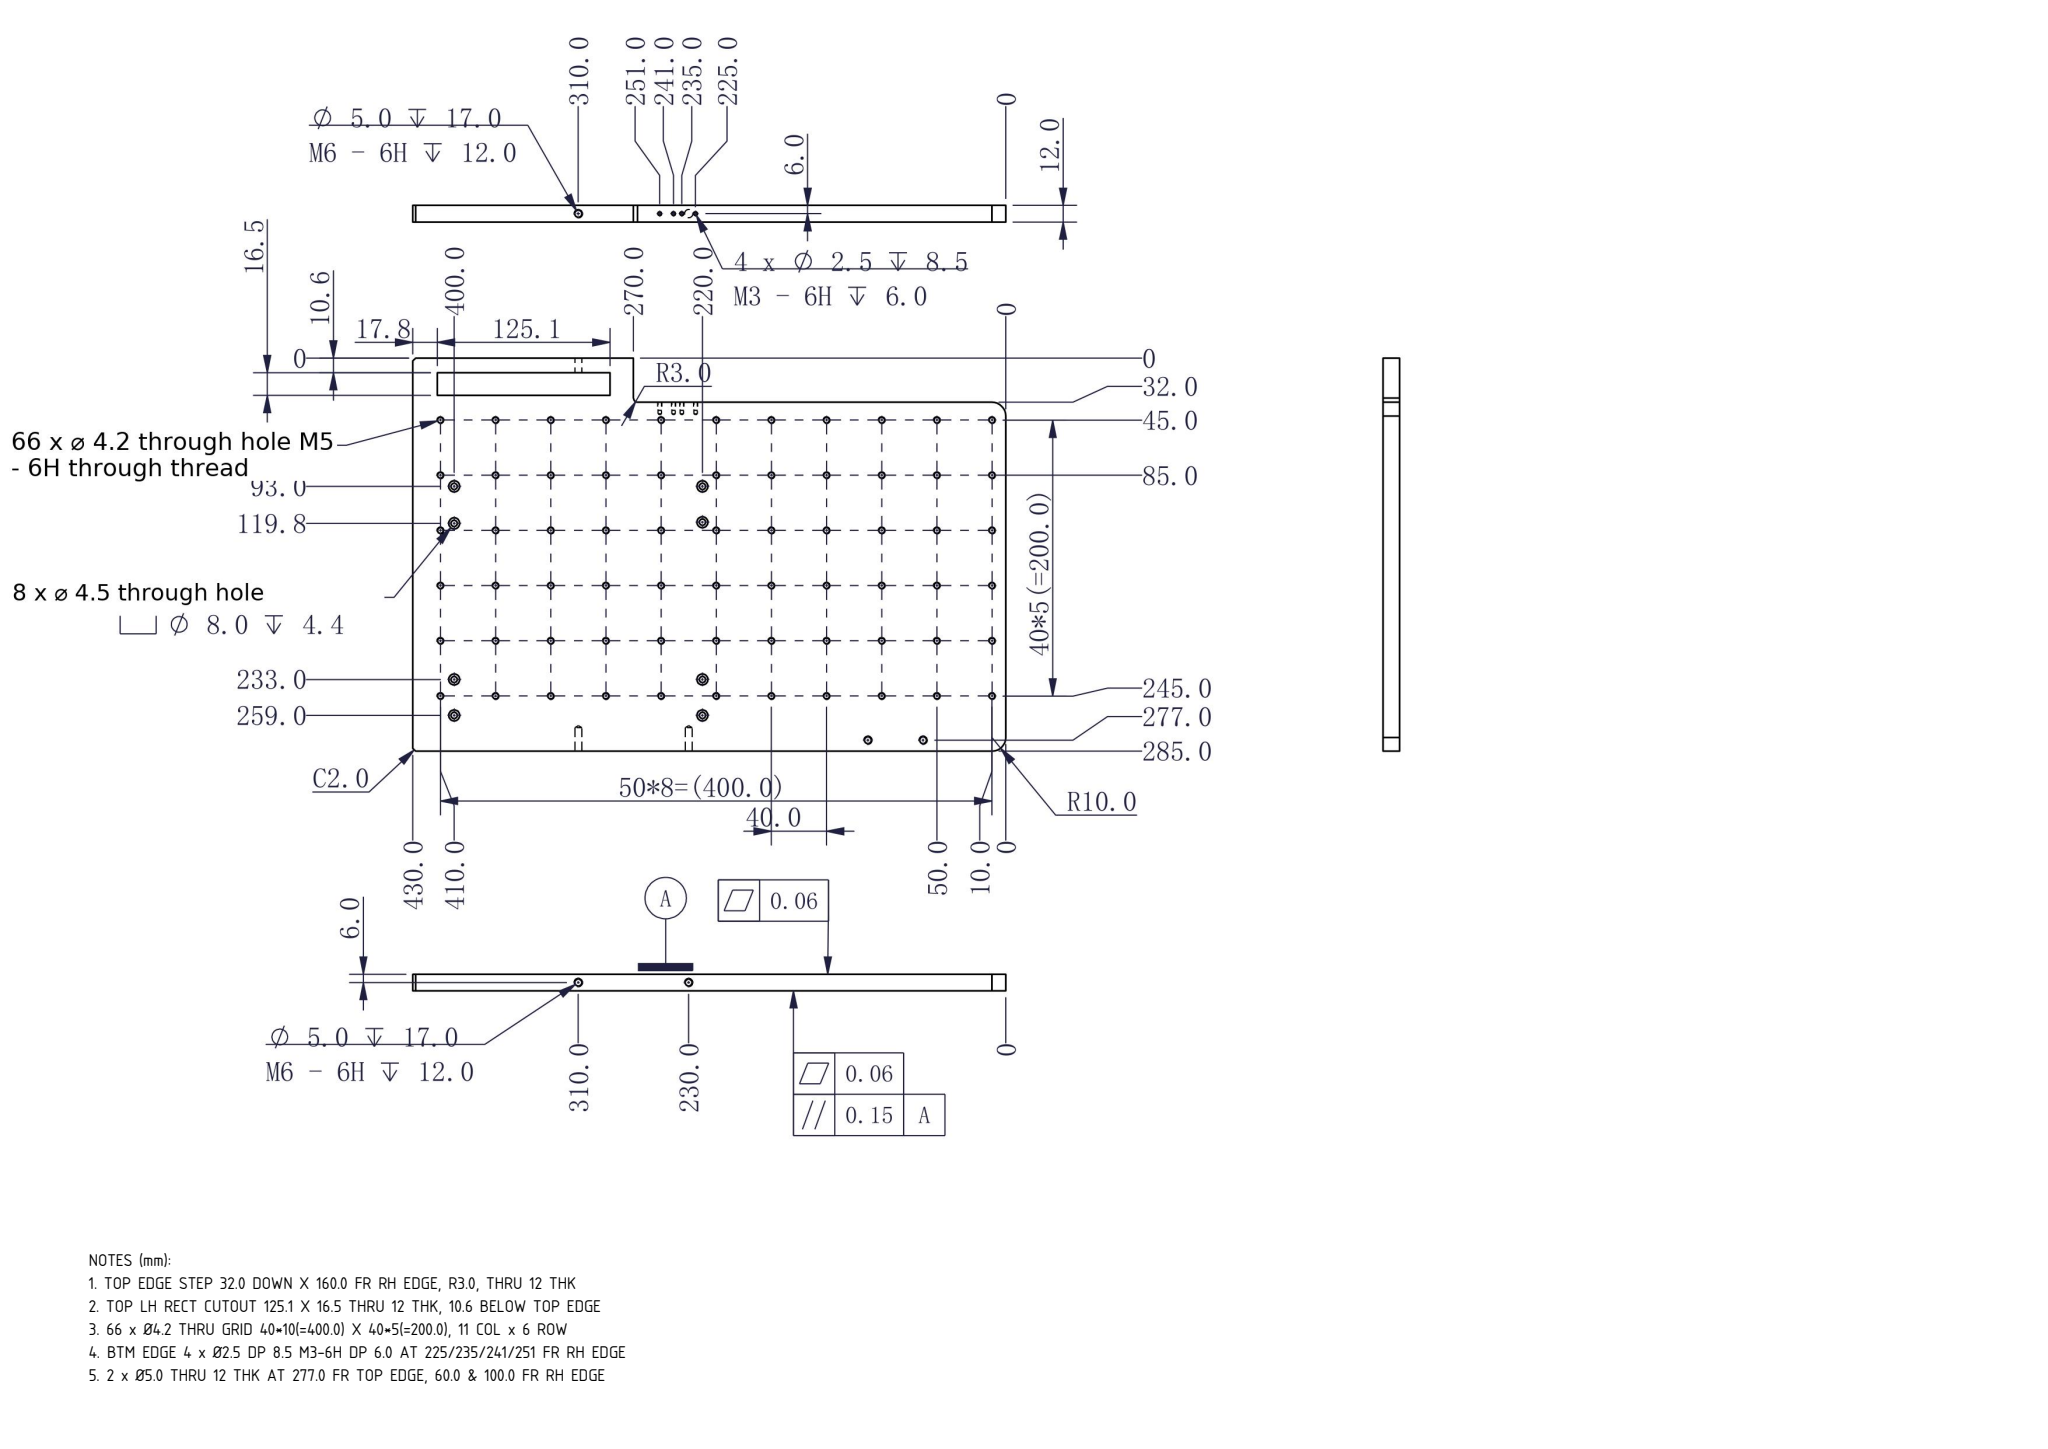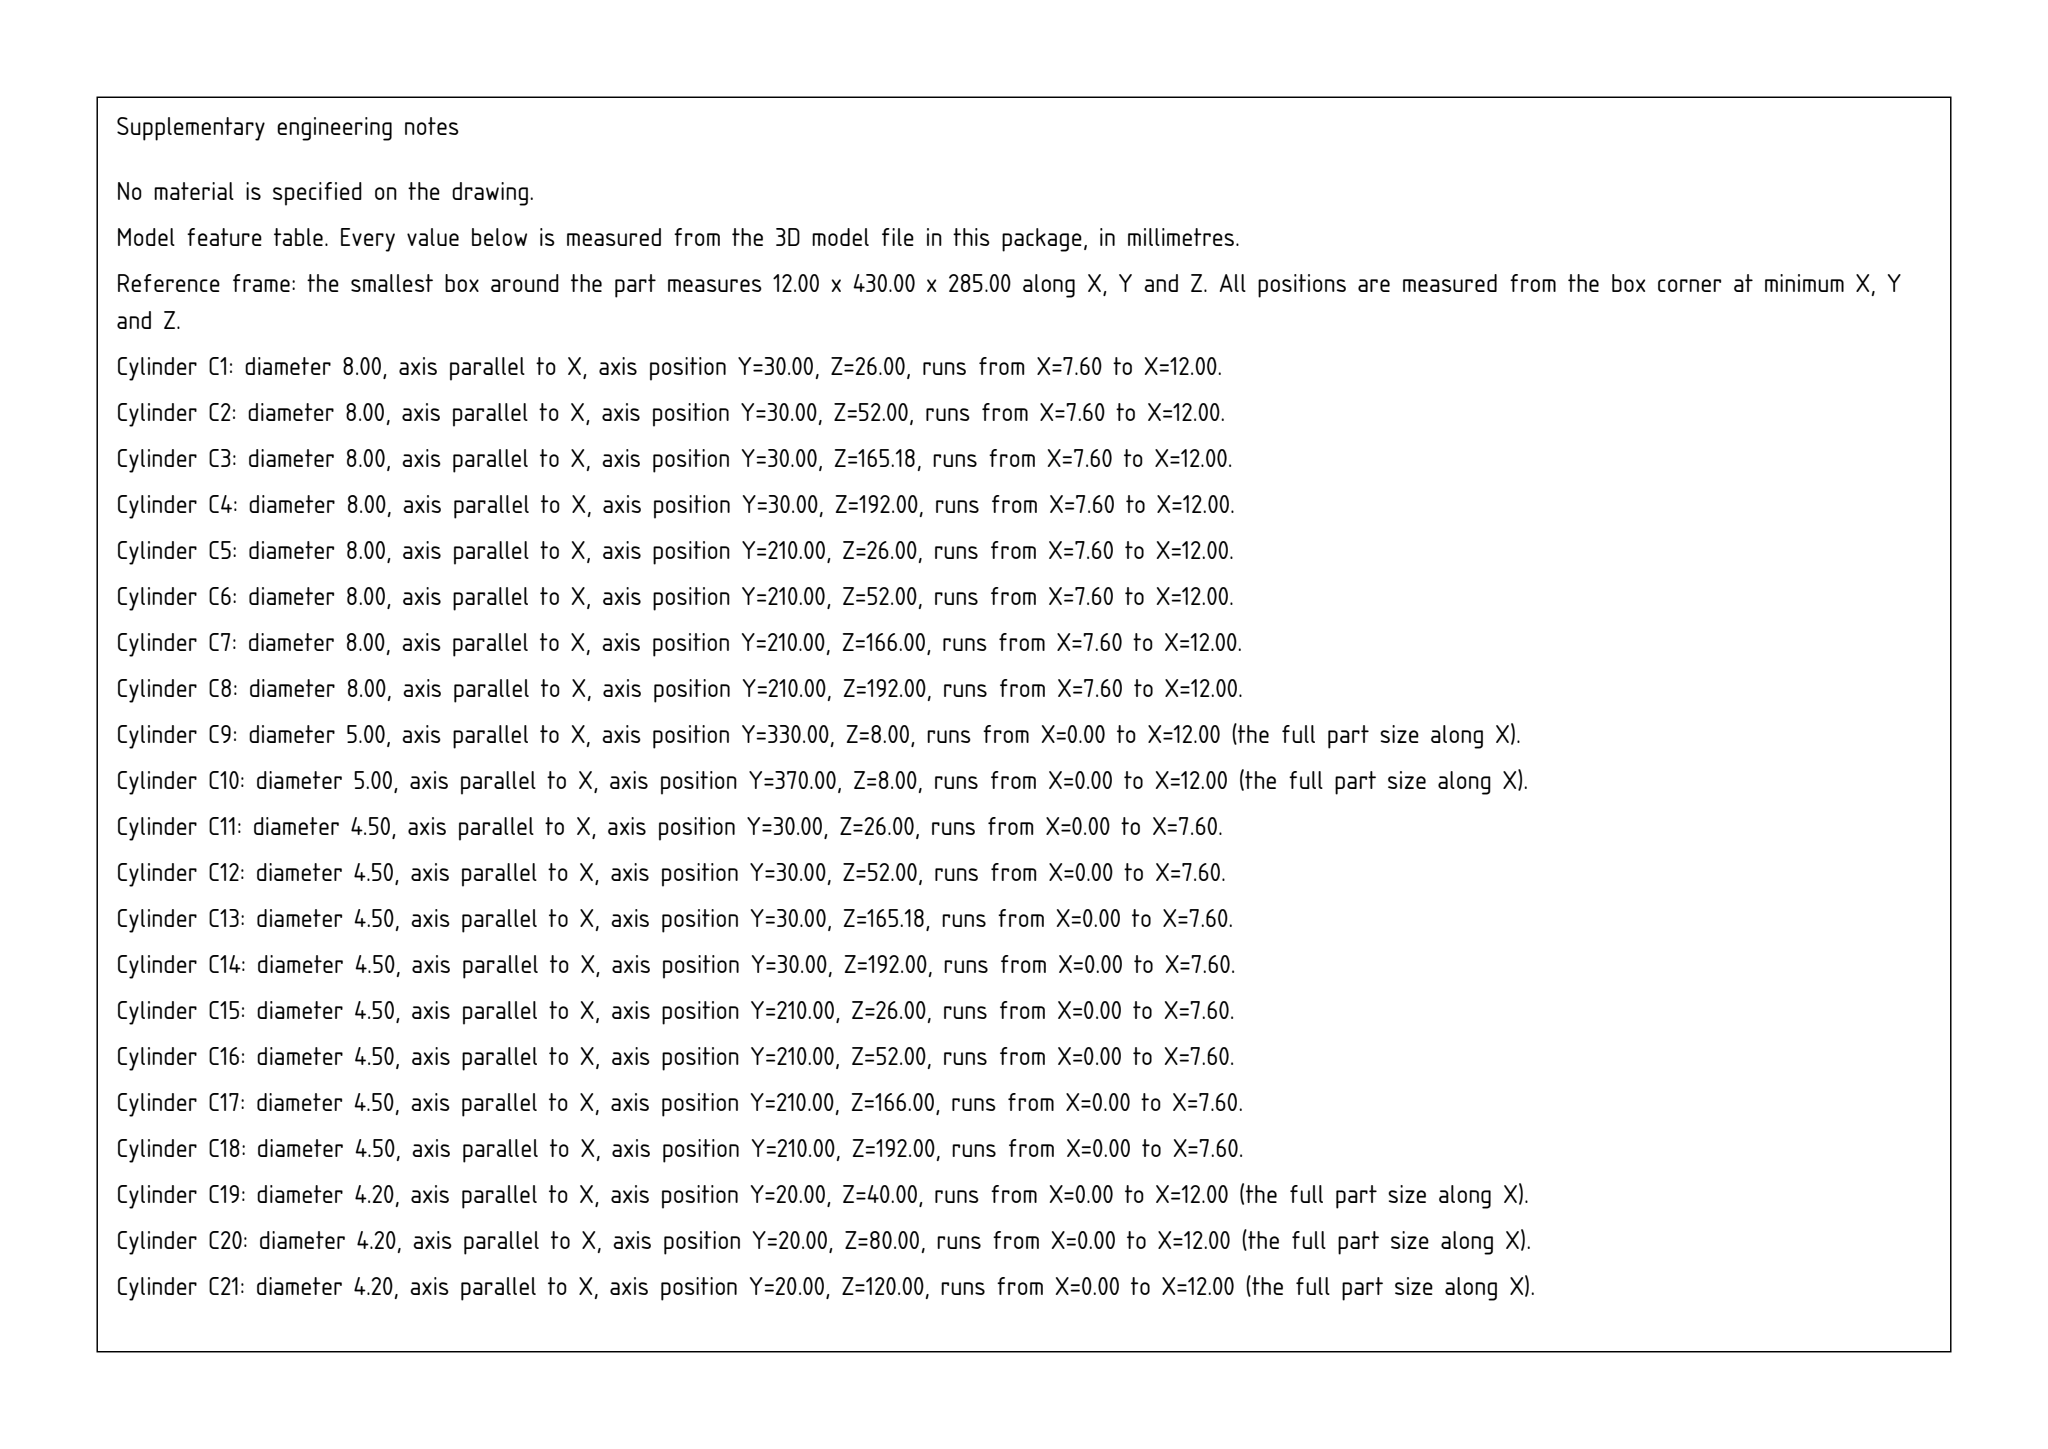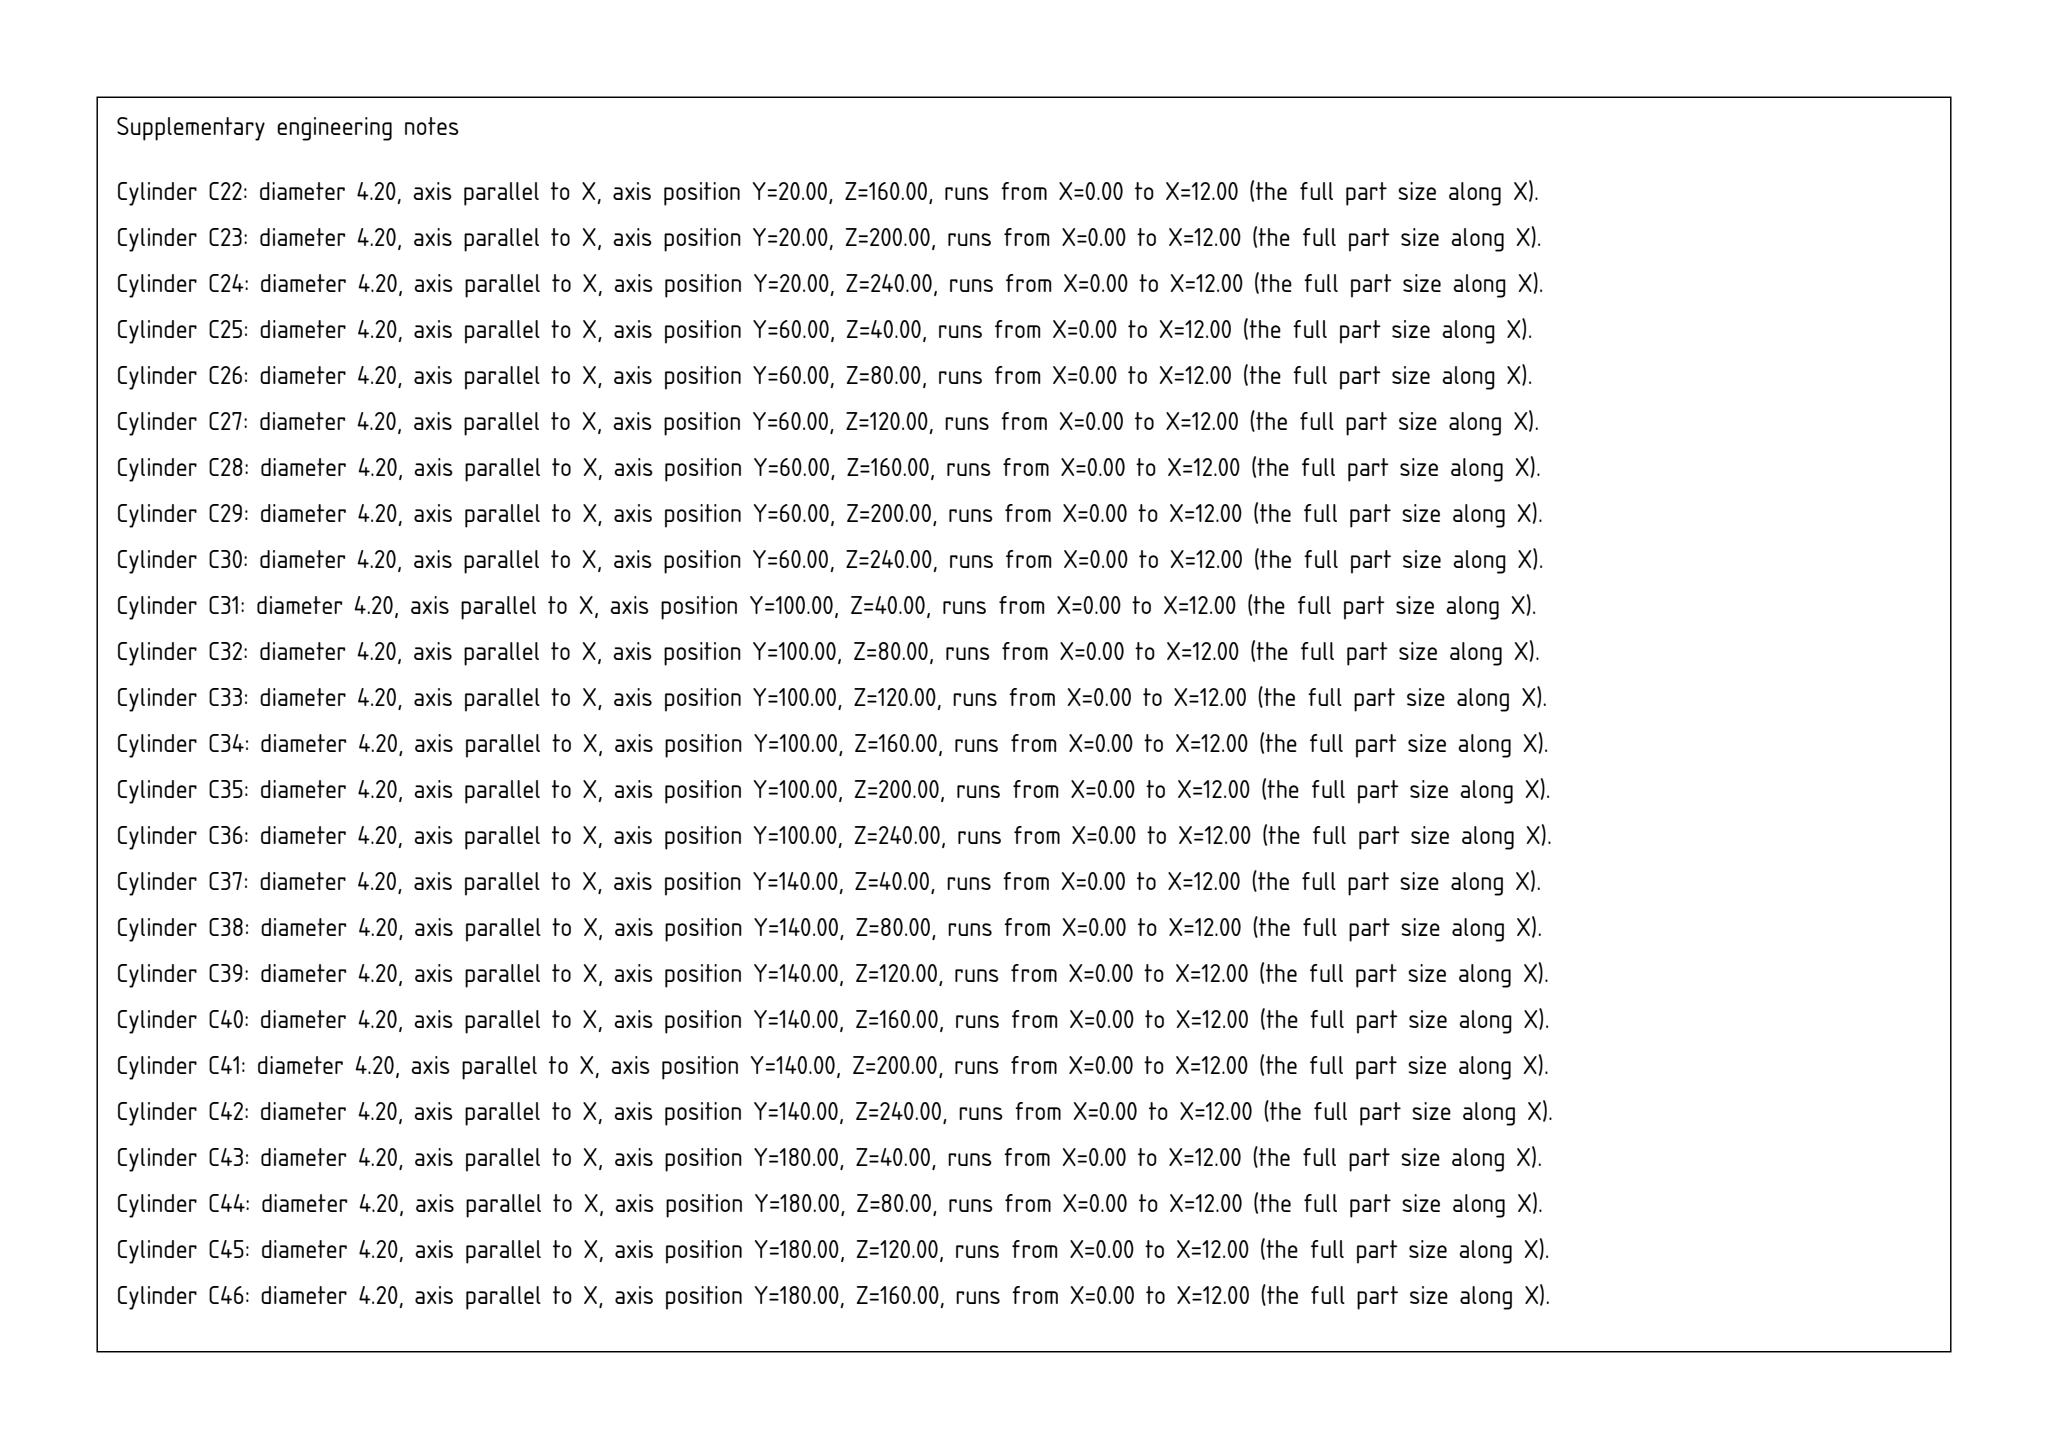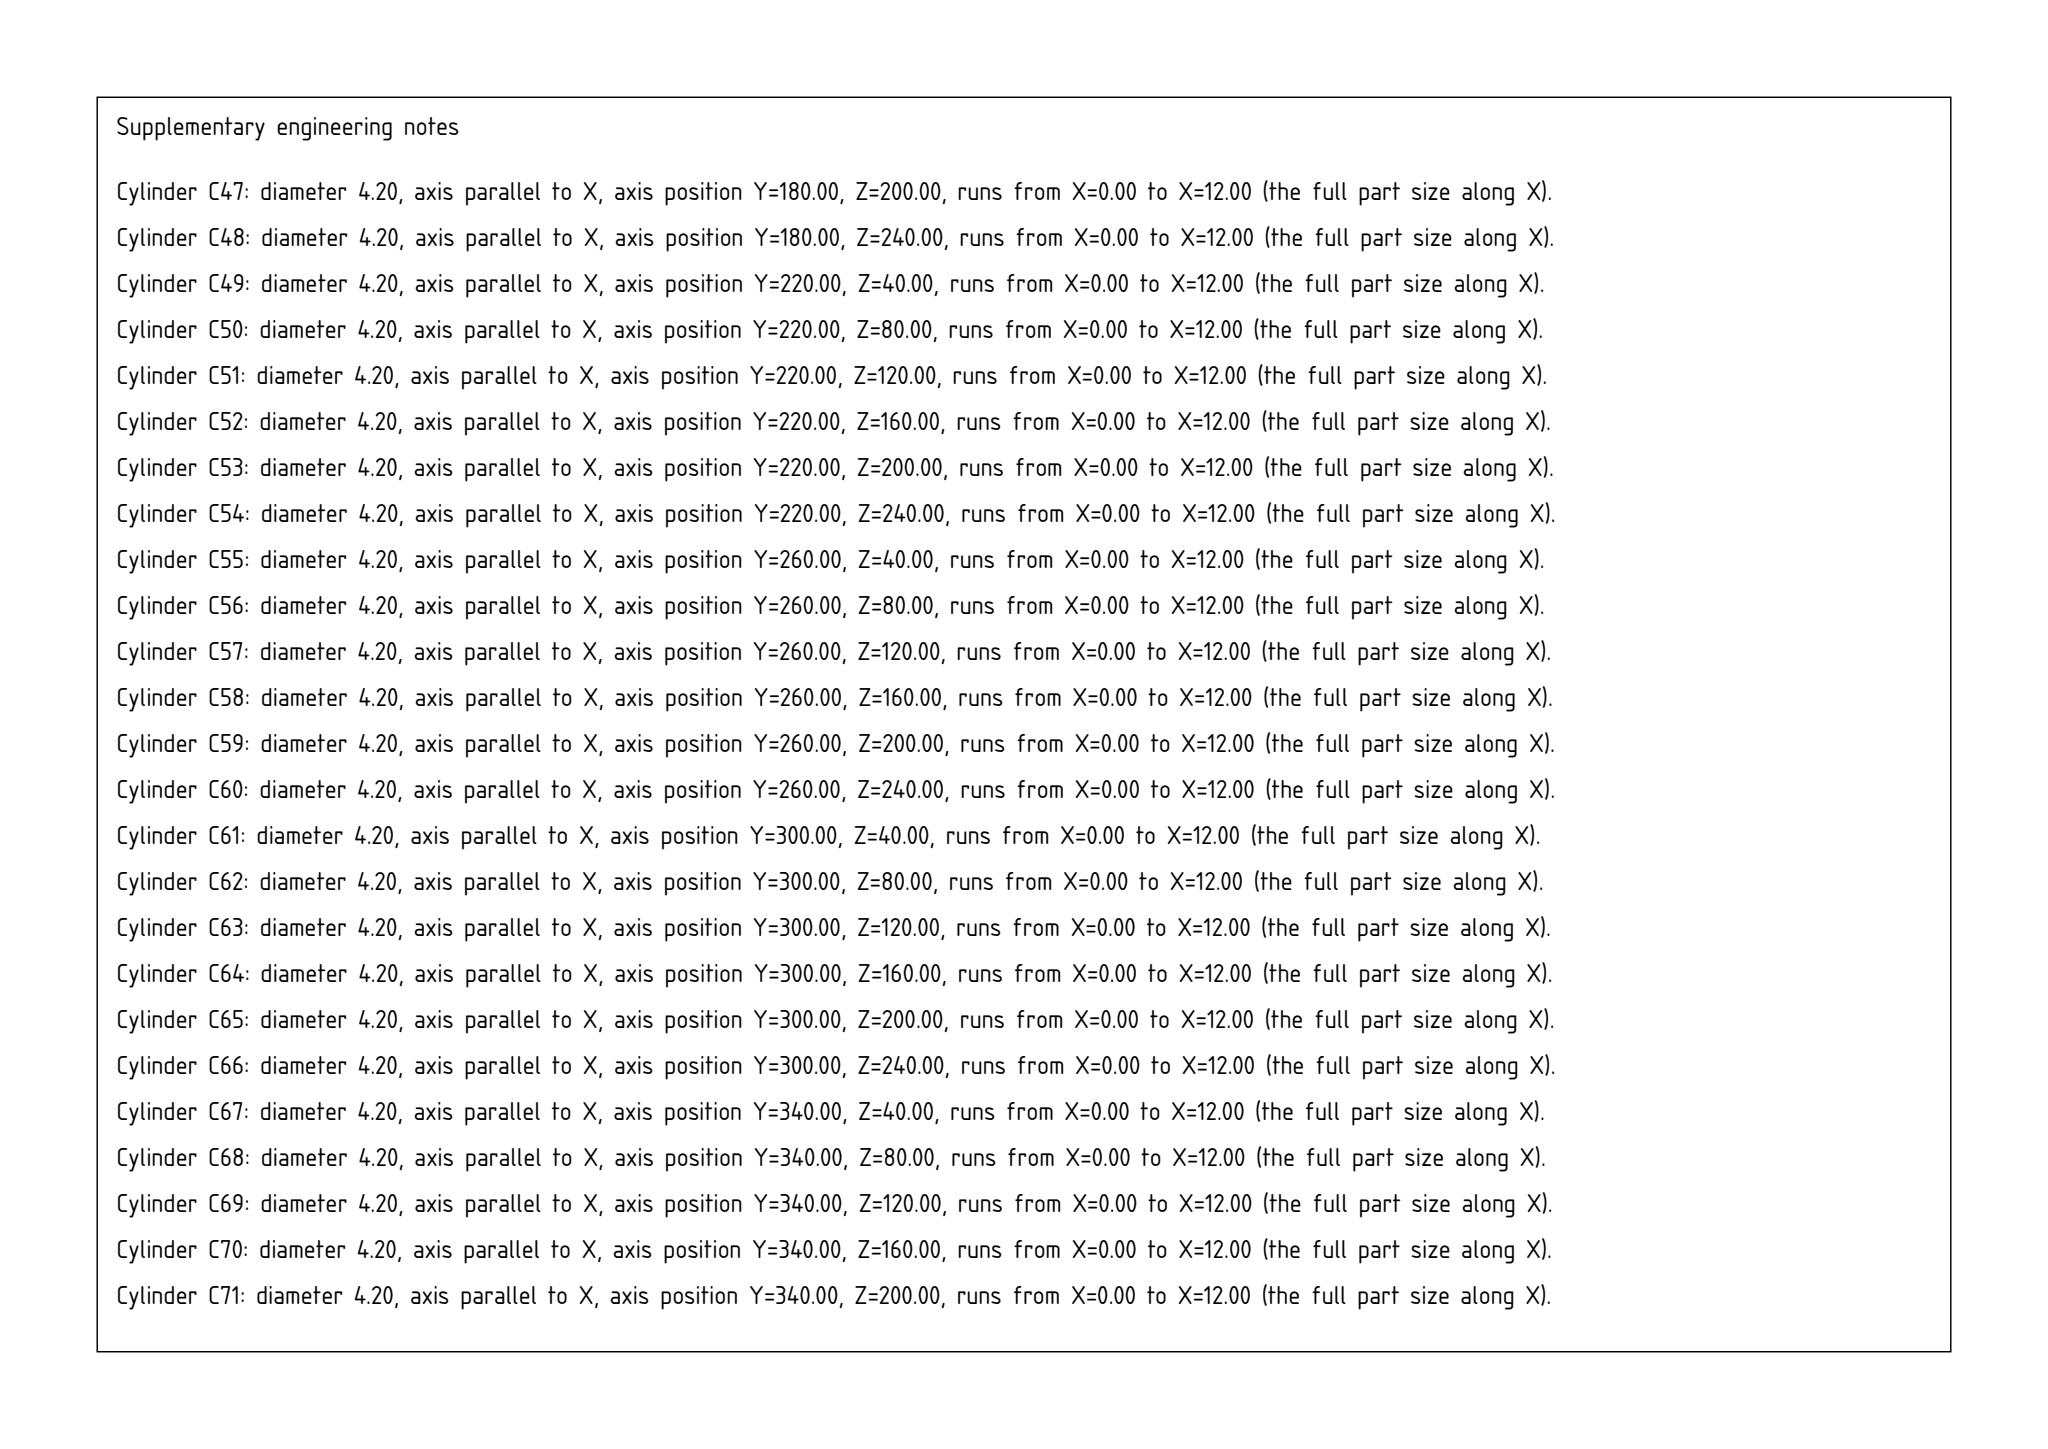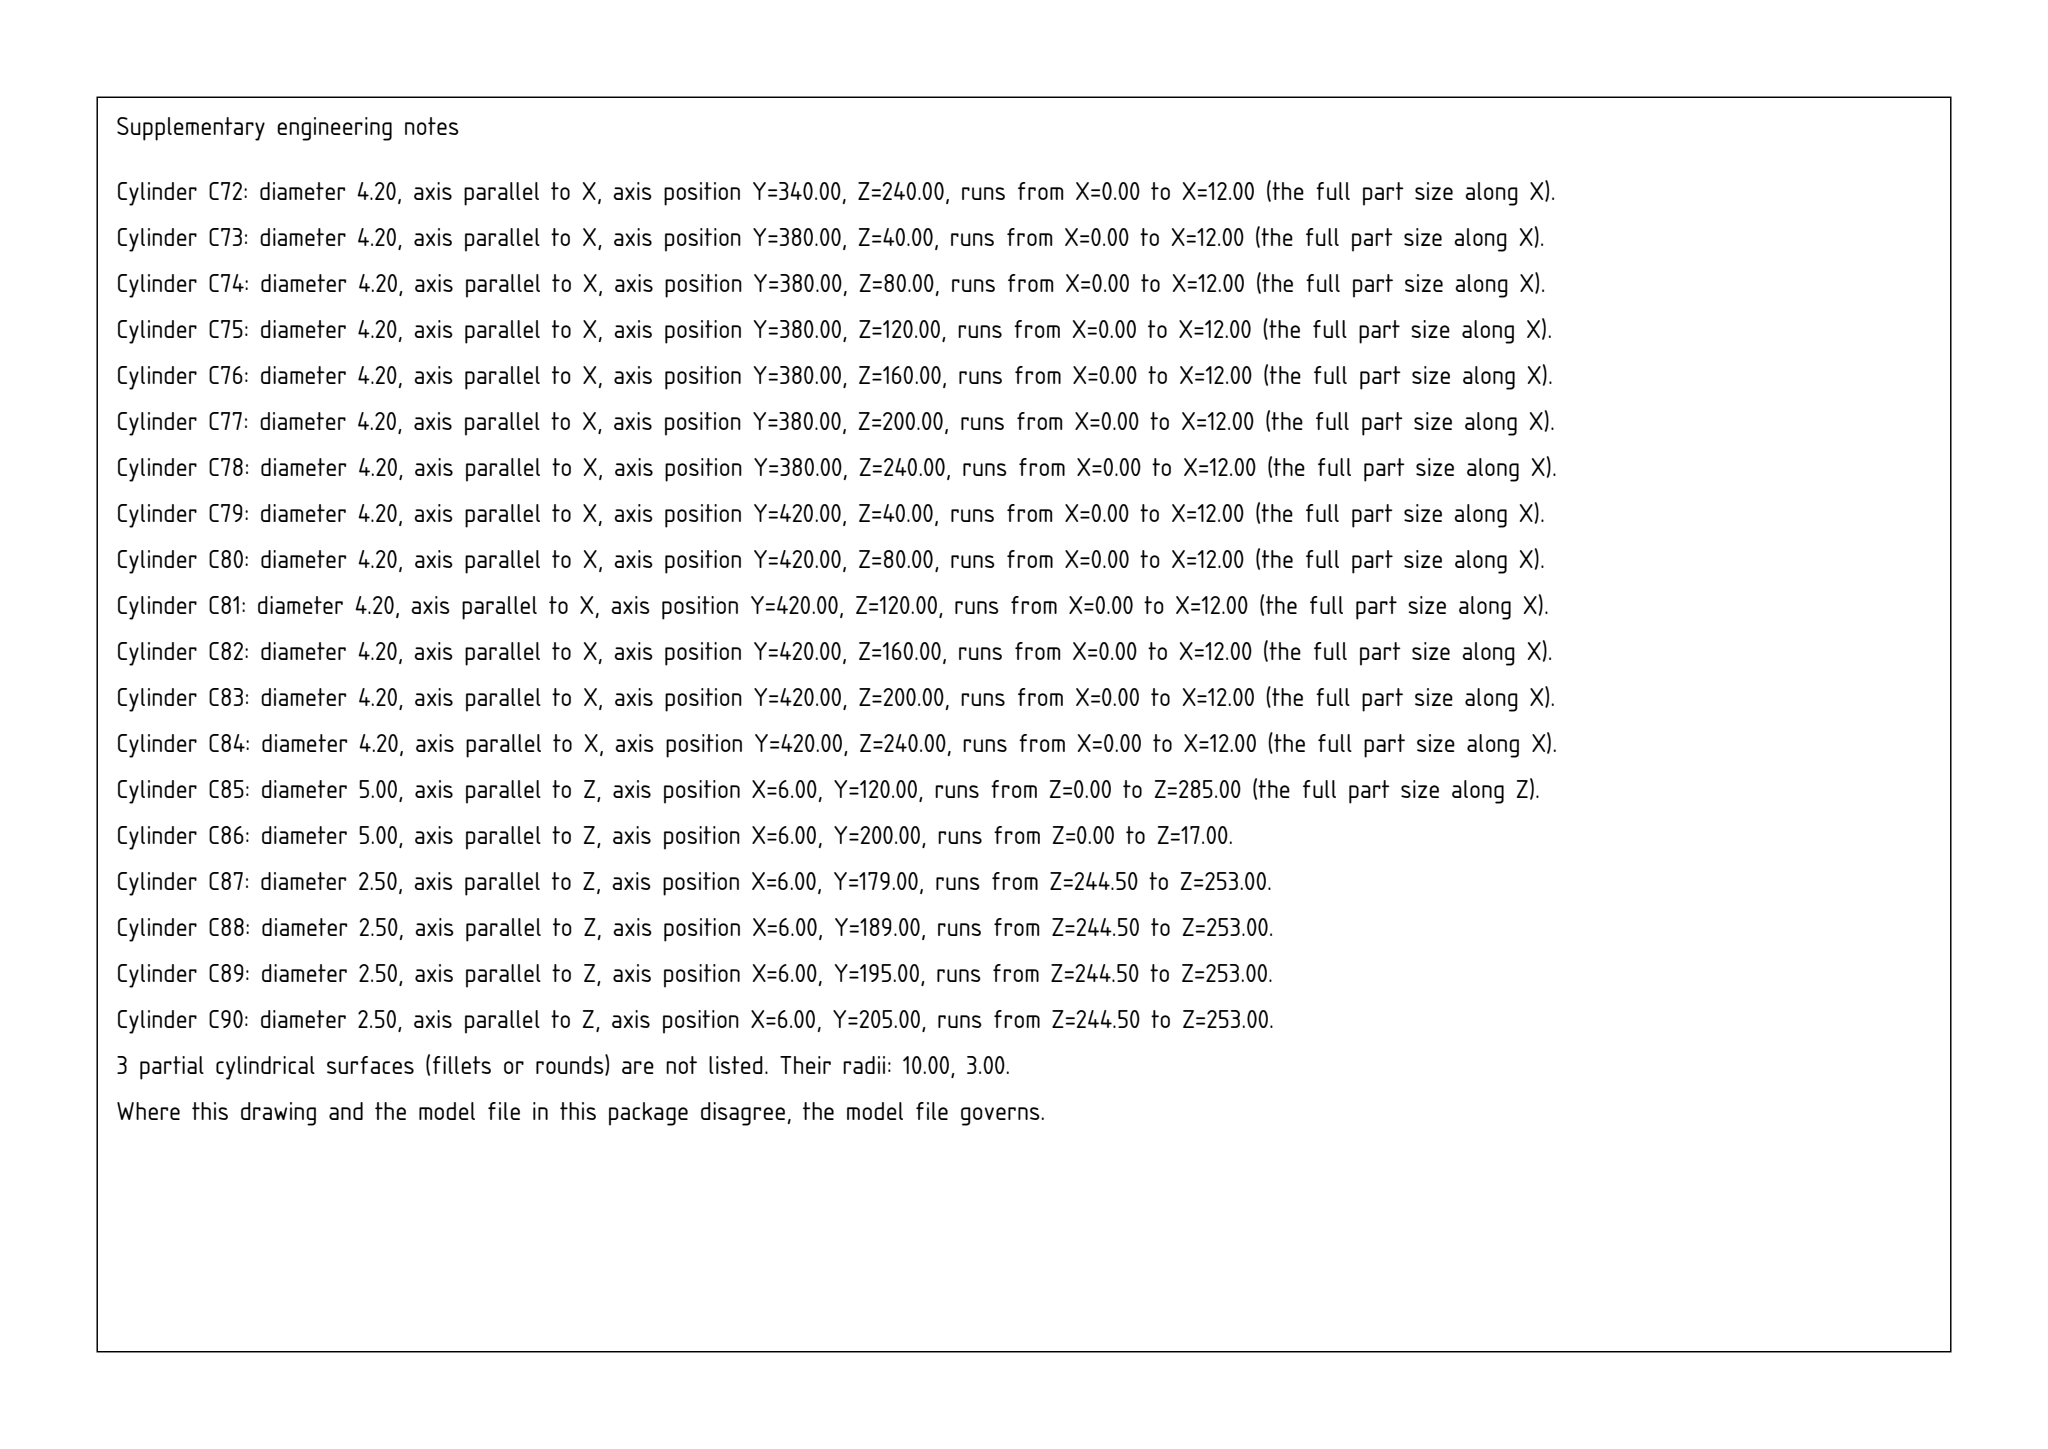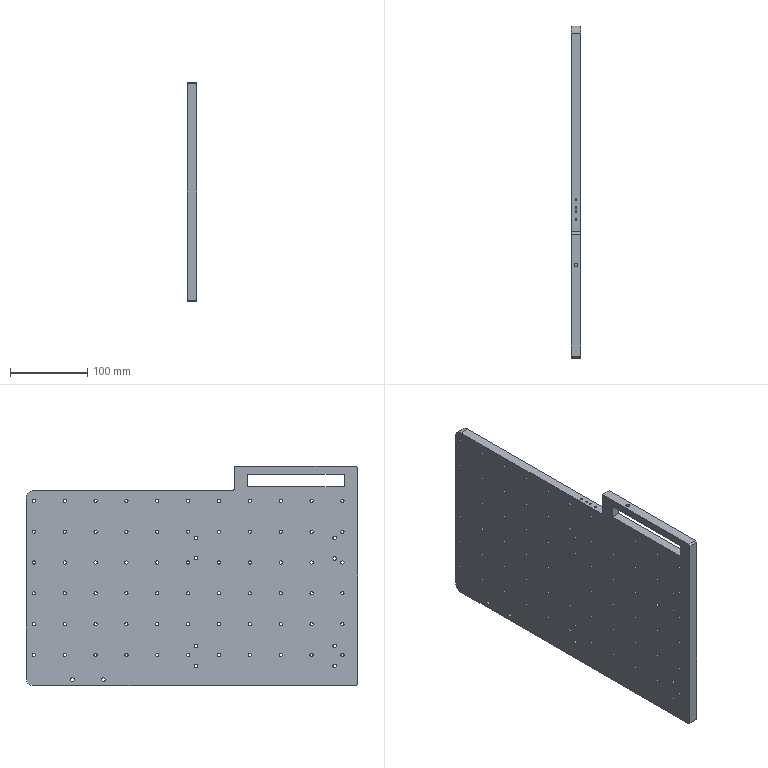Part | SolidWorks | mm | 1 solid | 219 faces | box 12 x 430 x 285 mm | volume 1326349 mm3 | cylinder 185 | plane 22 | cone 12 | commonest cylinder face diameters 4.2 x132 8 x16 4.5 x16 5 x10 2.5 x8 20 x2 6 x1
Drawing notes:
TOP EDGE STEP 32.0 DOWN X 160.0 FR RH EDGE, R3.0, THRU 12 THK | from the solid: y-plane 160.0; z-plane 253.0 (285-253=32.0); no intermediate x-plane so step is full 12 thk
TOP LH RECT CUTOUT 125.1 X 16.5 THRU 12 THK, 10.6 BELOW TOP EDGE | from the solid: y-planes 17.82 & 142.93 (=125.11); z-planes 274.42 & 257.91 (=16.51, 10.58 below top z=285); x-planes only 0/7.6/12
66 x Ø4.2 THRU GRID 40*10(=400.0) X 40*5(=200.0), 11 COL x 6 ROW | from the solid: Ø4.2 x-axis holes at y=20..420 step 40 (11) and z=40..240 step 40 (6) = 66; supersedes 50*8 pitch
BTM EDGE 4 x Ø2.5 DP 8.5 M3-6H DP 6.0 AT 225/235/241/251 FR RH EDGE | from the solid: Ø2.5 z-axis cyls len 8.5 at x=6.0, y=179/189/195/205; 430-y = 251/241/235/225 fr RH edge
2 x Ø5.0 THRU 12 THK AT 277.0 FR TOP EDGE, 60.0 & 100.0 FR RH EDGE | from the solid: Ø5.0 x-axis cyls len 12 at y=330 & 370, z=8.0; 285-8=277, 430-370=60, 430-330=100
build123d program:
from build123d import *

# Parameters (mm, degrees)
SKETCH1_W                                       = 285
SKETCH1_H                                       = 430
BOSS_EXTRUDE1_DEPTH                             = 12
CHAMFER1_SIZE                                   = 2
SKETCH11_W                                      = 32
SKETCH11_H                                      = 270
CUT_EXTRUDE2_DEPTH                              = 259.216
FILLET1_R                                       = 3
LPATTERN1_COUNT                                 = 2
LPATTERN1_PITCH                                 = 80
M4_HEX_SOCKET_HEAD_CAP_SCREW_CBORE1_D           = 4.5
M4_HEX_SOCKET_HEAD_CAP_SCREW_CBORE1_CBORE_D     = 8
M4_HEX_SOCKET_HEAD_CAP_SCREW_CBORE1_CBORE_DEPTH = 4.4
M6_TAPPED_HOLE3_D                               = 5
FILLET2_R                                       = 10
FILLET3_R                                       = 10
M5_TAPPED_HOLE1_D                               = 4.2
LPATTERN2_COUNT                                 = 11
LPATTERN2_PITCH                                 = 40
LPATTERN2_COUNT_DIR2                            = 6
LPATTERN2_PITCH_DIR2                            = 40
M3_TAPPED_HOLE1_D                               = 2.5
M3_TAPPED_HOLE1_DEPTH                           = 8.5
M3_TAPPED_HOLE1_TIP                             = 0.7511
SKETCH22_W                                      = 16.507
SKETCH22_H                                      = 125.118
CUT_EXTRUDE3_DEPTH                              = 104


with BuildPart() as part:
    # Sketch1 → Boss-Extrude1 (new body)
    with BuildSketch(Plane(origin=(0, 0, 0), x_dir=(0, 0, -1), z_dir=(1, 0, 0))):
        Rectangle(SKETCH1_W, SKETCH1_H)
    extrude(amount=BOSS_EXTRUDE1_DEPTH)

    # Chamfer1
    chamfer1_edges = [part.edges().sort_by_distance(p)[0] for p in [
        (6, -215, -142.5),
        (6, -215, 142.5),
        (6, 215, 142.5),
    ]]
    chamfer(chamfer1_edges, length=CHAMFER1_SIZE)

    # Sketch8 → M6 Tapped Hole1 (revolve, cut)
    with BuildSketch(Plane(origin=(6, -15, 142.5), x_dir=(0, -1, 0), z_dir=(1, 0, 0))):
        Polygon((0, 0), (0, 18.502), (2.5, 17), (2.5, 0), align=None)
    m6_tapped_hole1 = revolve(axis=Axis((6, -15, 148.85), (0, 0, -1)), mode=Mode.SUBTRACT)

    # Mirror1: M6 Tapped Hole1 across plane
    add(m6_tapped_hole1.mirror(Plane.XY), mode=Mode.SUBTRACT)

    # Sketch11 → Cut-Extrude2 (cut, through all)
    with BuildSketch(Plane(origin=(12, 0, 0), x_dir=(0, 0, -1), z_dir=(1, 0, 0))):
        with Locations((-126.5, 80)):
            Rectangle(SKETCH11_W, SKETCH11_H)
    extrude(amount=-CUT_EXTRUDE2_DEPTH, mode=Mode.SUBTRACT)

    # Fillet1
    fillet1_edges = [part.edges().sort_by_distance(p)[0] for p in [
        (6, -55, 110.5),
    ]]
    fillet(fillet1_edges, radius=FILLET1_R)

    # LPattern1: M6 Tapped Hole1 ×2
    with Locations(*[(0, -i * LPATTERN1_PITCH, 0) for i in range(1, LPATTERN1_COUNT)]):
        add(m6_tapped_hole1, mode=Mode.SUBTRACT)

    # LPattern1 copy 1 sketch → LPattern1 copy 1 (revolve, cut)
    with BuildSketch(Plane(origin=(6, -95, -142.5), x_dir=(0, -1, 0), z_dir=(1, 0, 0))):
        Polygon((0, 0), (0, -18.502), (2.5, -17), (2.5, 0), align=None)
    revolve(axis=Axis((6, -95, -148.85), (0, 0, -1)), mode=Mode.SUBTRACT)

    # M4 Hex Socket Head Cap Screw CBORE1 (through all)
    with Locations(Plane(origin=(12, 0, 0), x_dir=(0, 0, -1), z_dir=(1, 0, 0))):
        with Locations((116.5, -185), (90.5, -185), (-22.675, -185), (-49.5, -185), (116.5, -5), (90.5, -5), (-23.5, -5), (-49.5, -5)):
            CounterBoreHole(M4_HEX_SOCKET_HEAD_CAP_SCREW_CBORE1_D / 2, M4_HEX_SOCKET_HEAD_CAP_SCREW_CBORE1_CBORE_D / 2, M4_HEX_SOCKET_HEAD_CAP_SCREW_CBORE1_CBORE_DEPTH)

    # M6 Tapped Hole3 (through all)
    with Locations(Plane(origin=(12, 0, 0), x_dir=(0, 0, -1), z_dir=(1, 0, 0))):
        with Locations((134.5, 115), (134.5, 155)):
            Hole(M6_TAPPED_HOLE3_D / 2)

    # Fillet2
    fillet2_edges = [part.edges().sort_by_distance(p)[0] for p in [
        (6, 215, 110.5),
    ]]
    fillet(fillet2_edges, radius=FILLET2_R)

    # Fillet3
    fillet3_edges = [part.edges().sort_by_distance(p)[0] for p in [
        (6, 215, -142.5),
    ]]
    fillet(fillet3_edges, radius=FILLET3_R)

    # M5 Tapped Hole1 (through all)
    with Locations(Plane(origin=(12, 0, 0), x_dir=(0, 0, -1), z_dir=(1, 0, 0))):
        with Locations((102.5, -195)):
            m5_tapped_hole1 = Hole(M5_TAPPED_HOLE1_D / 2)

    # LPattern2: M5 Tapped Hole1 11 × 6
    with Locations(*[(0, i * LPATTERN2_PITCH, j * LPATTERN2_PITCH_DIR2) for i in range(LPATTERN2_COUNT) for j in range(LPATTERN2_COUNT_DIR2) if (i, j) != (0, 0)]):
        add(m5_tapped_hole1, mode=Mode.SUBTRACT)

    # M3 Tapped Hole1
    with Locations(Plane.XY.offset(110.5)):
        with Locations((6, -36), (6, -26), (6, -20), (6, -10)):
            Hole(M3_TAPPED_HOLE1_D / 2, depth=M3_TAPPED_HOLE1_DEPTH)
            with Locations((0, 0, -(M3_TAPPED_HOLE1_DEPTH + M3_TAPPED_HOLE1_TIP / 2))):  # 118° drill point
                Cone(0, M3_TAPPED_HOLE1_D / 2, M3_TAPPED_HOLE1_TIP, mode=Mode.SUBTRACT)

    # Sketch22 → Cut-Extrude3 (cut)
    with BuildSketch(Plane(origin=(12, 0, 0), x_dir=(0, 0, -1), z_dir=(1, 0, 0))):
        with Locations((-123.662, -134.624)):
            Rectangle(SKETCH22_W, SKETCH22_H)
    extrude(amount=-CUT_EXTRUDE3_DEPTH, mode=Mode.SUBTRACT)


solid = part.part